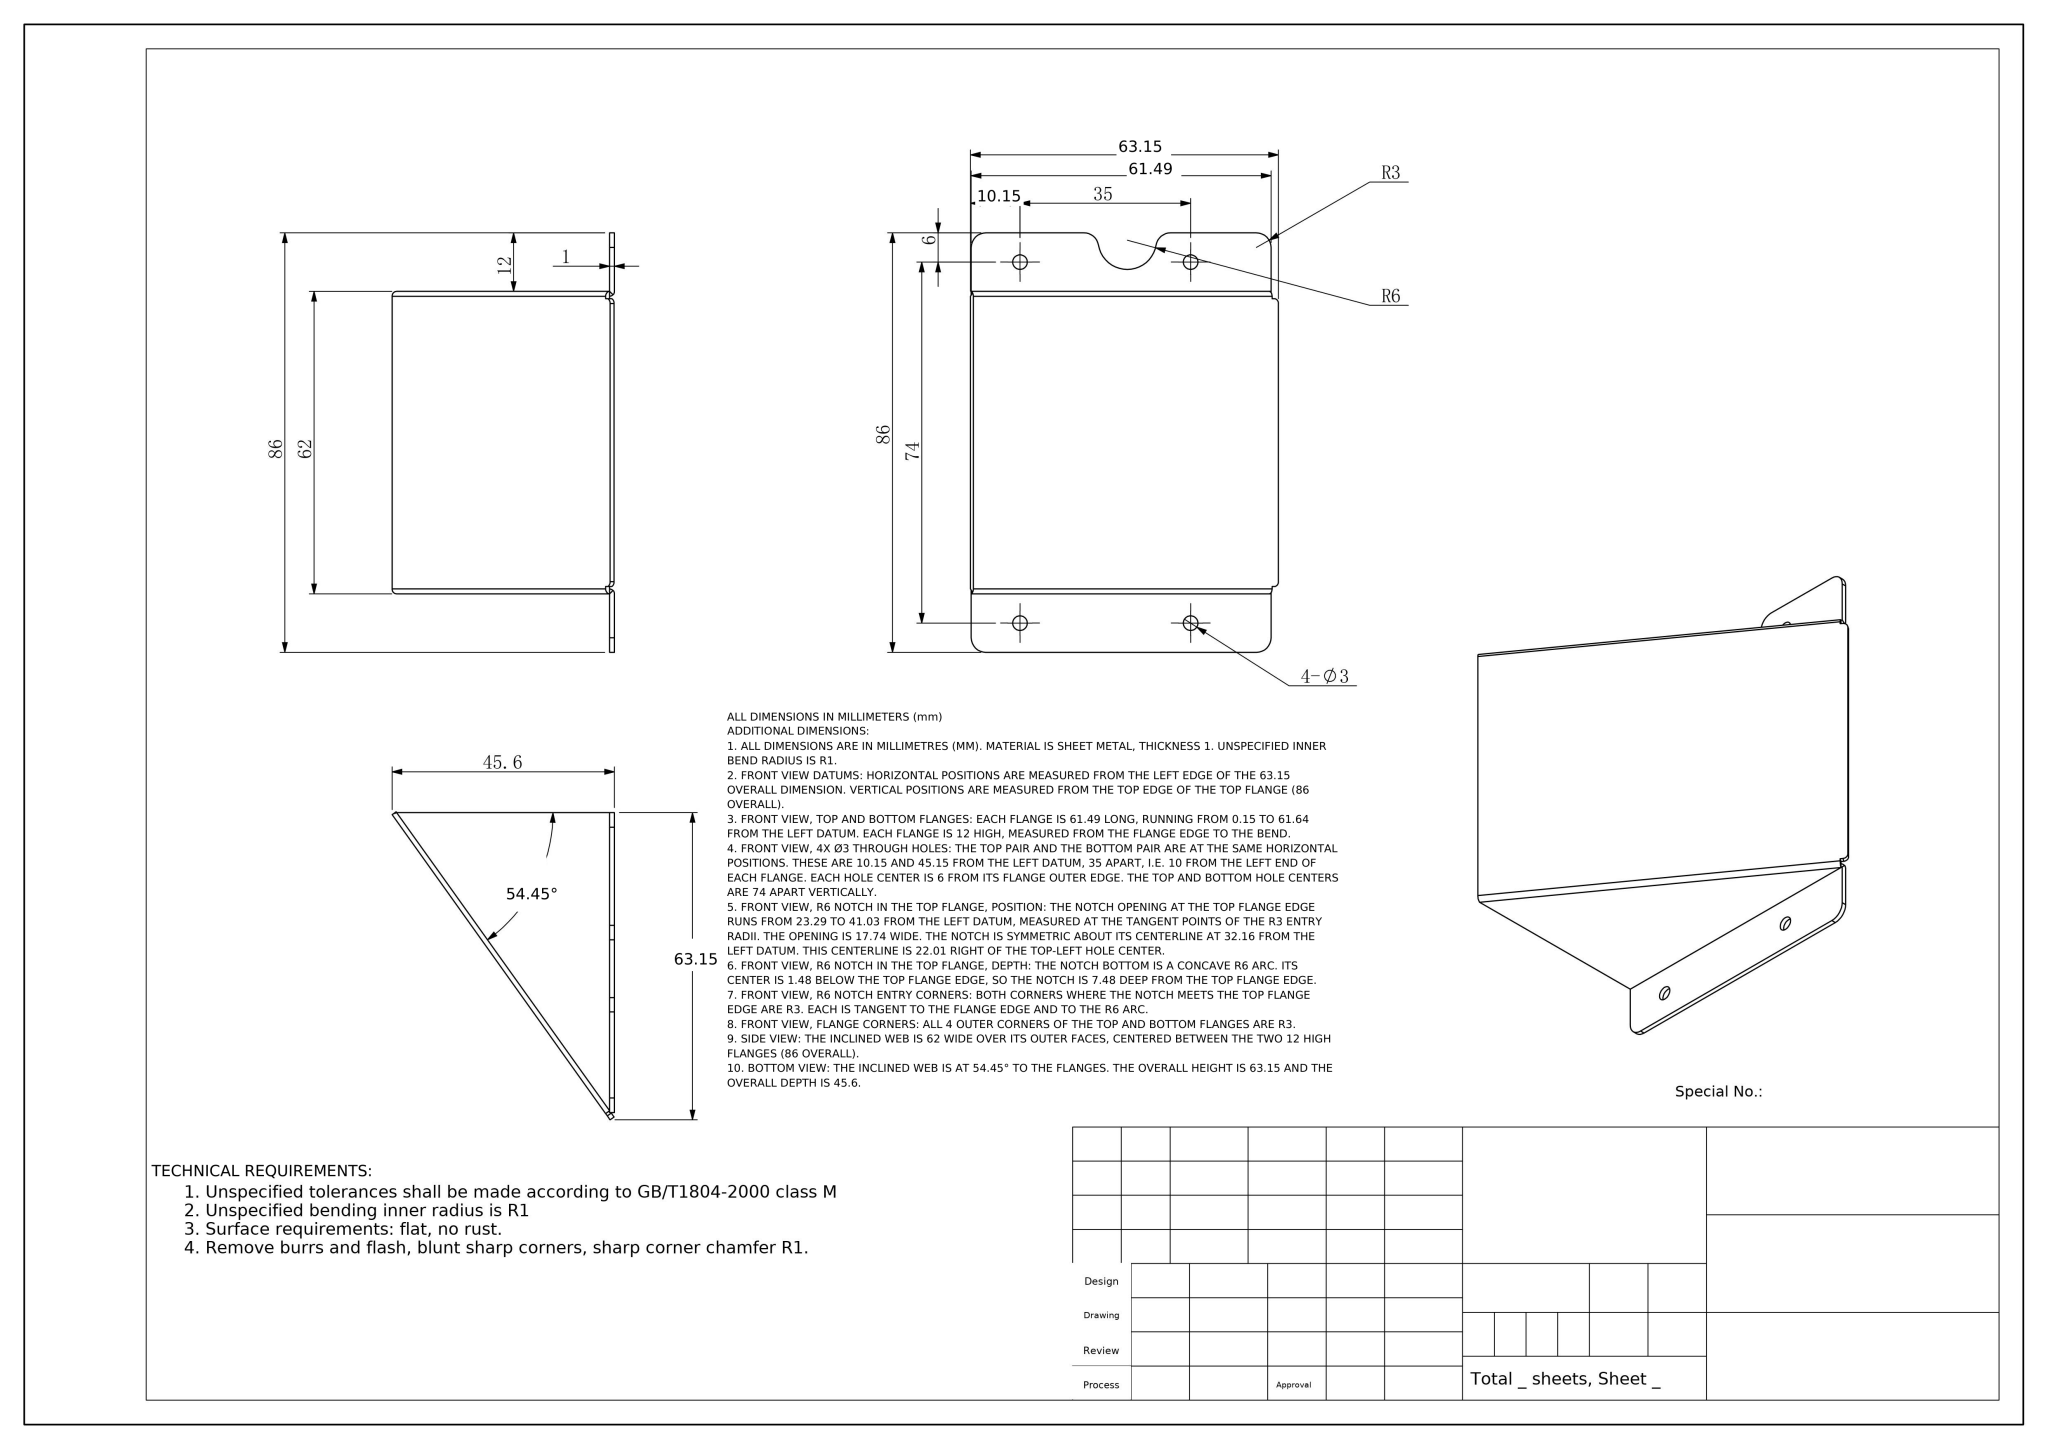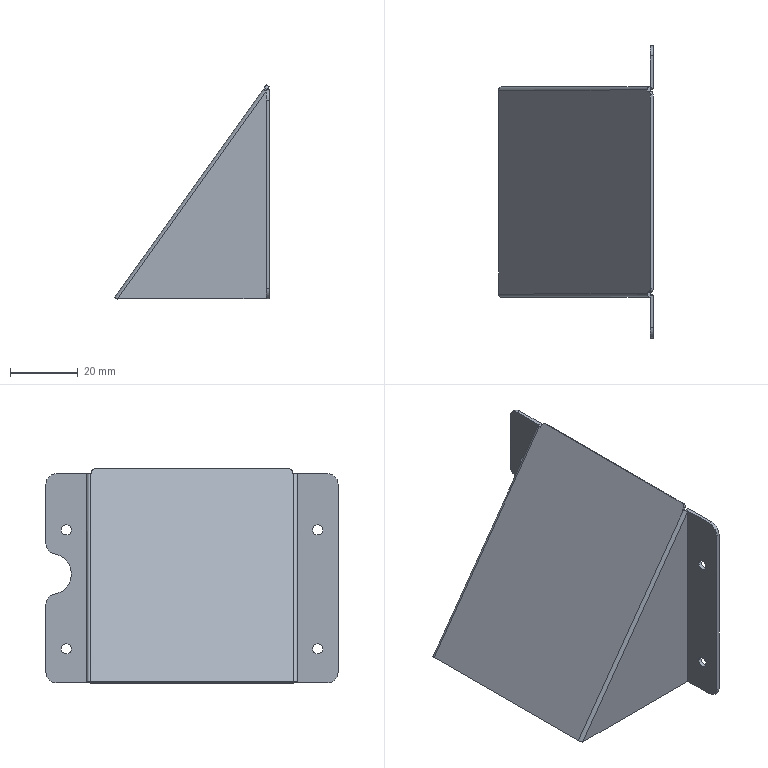Part | NX | mm | 1 solid | 53 faces | box 45.6 x 86 x 63.15 mm | volume 8859 mm3 | cylinder 26 | plane 23 | spline 4 | commonest cylinder face diameters 3 x8 6 x6 2.004 x4 0.004 x4 12 x2 2 x2